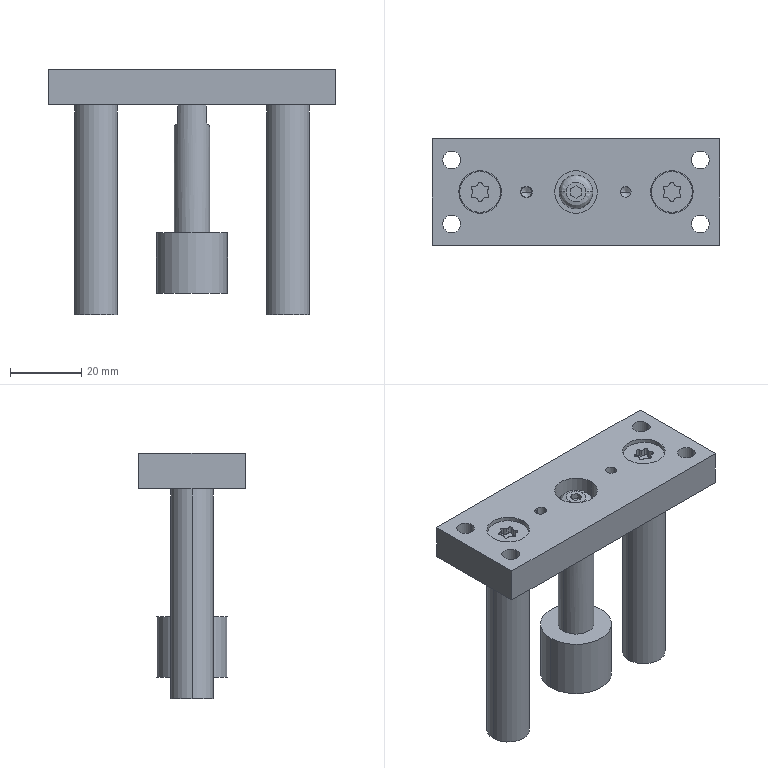Component | SolidWorks | 1-VASP2004STG-M-PlateGuideRod_default-1 | 1 solid | 114 faces | volume 44112 mm3 | cylinder 75 | plane 33 | cone 4 | spline 2 | commonest cylinder face diameters 2 x24 1.12 x16 12 x10 5 x8 3 x7 11.5 x4 10 x2 20 x2